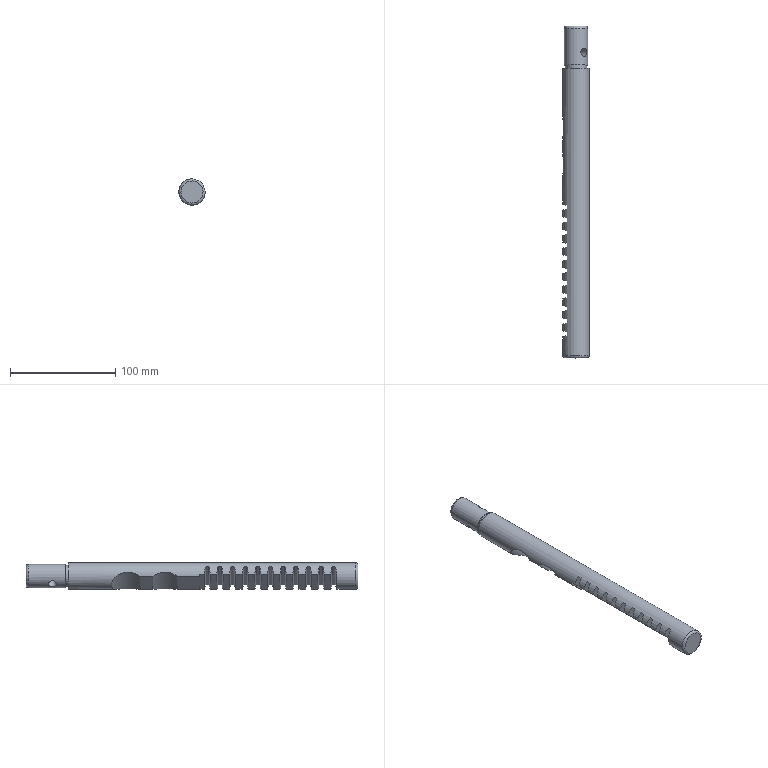Component | NX | MODEL1 | 1 solid | 60 faces | volume 125319 mm3 | plane 52 | cylinder 6 | torus 2 | commonest cylinder face diameters 45 x2 25 x1 22 x1 20 x1 8 x1